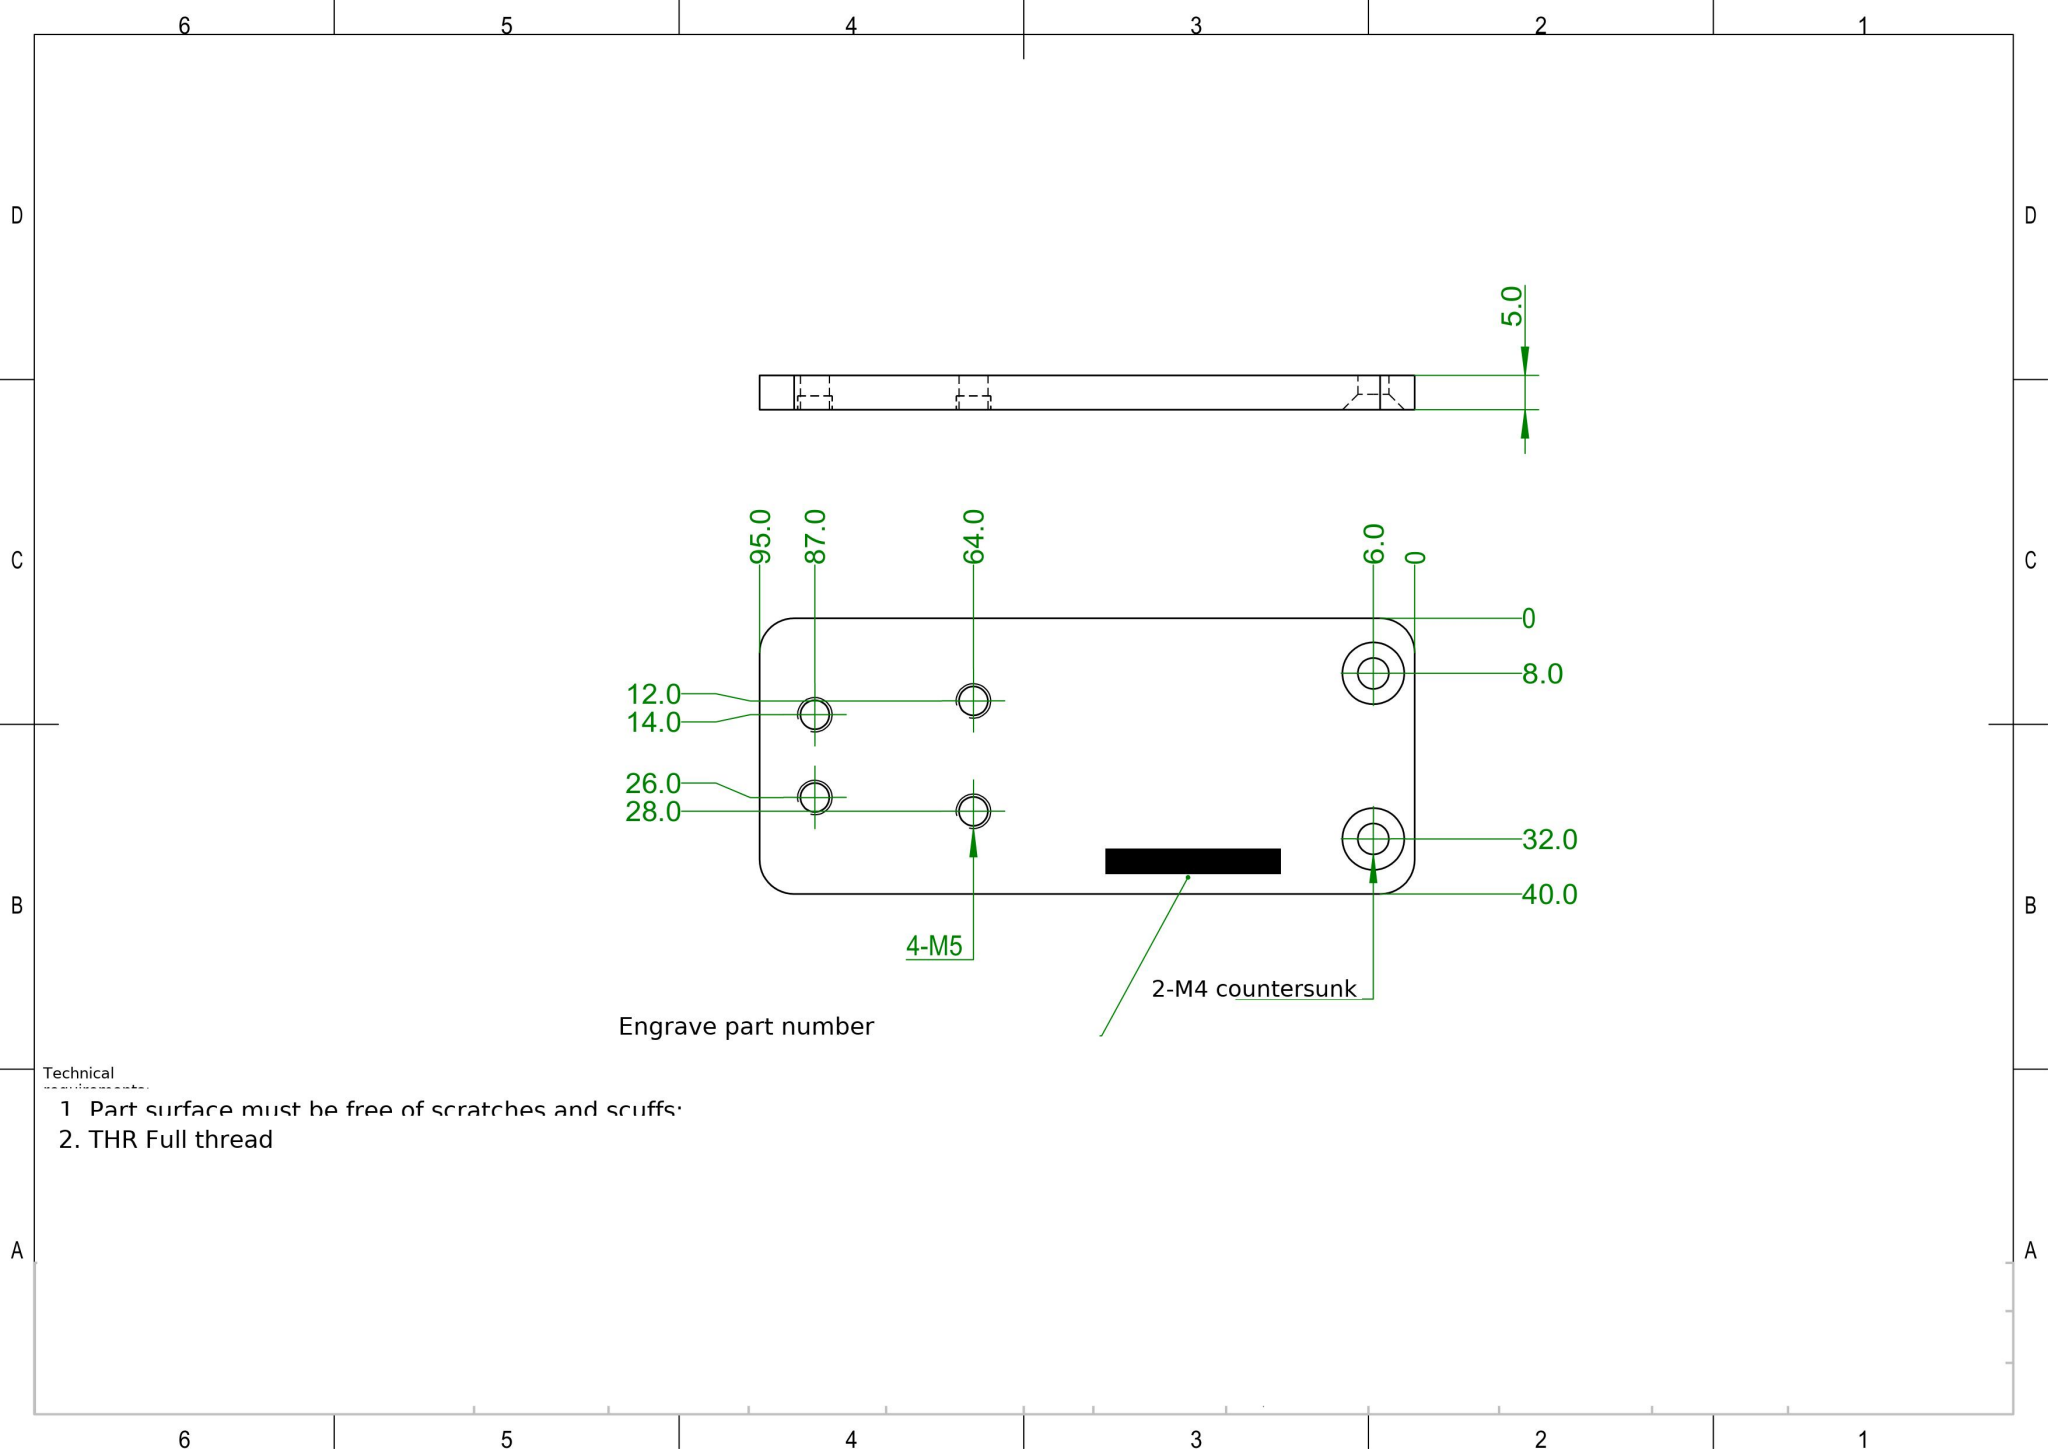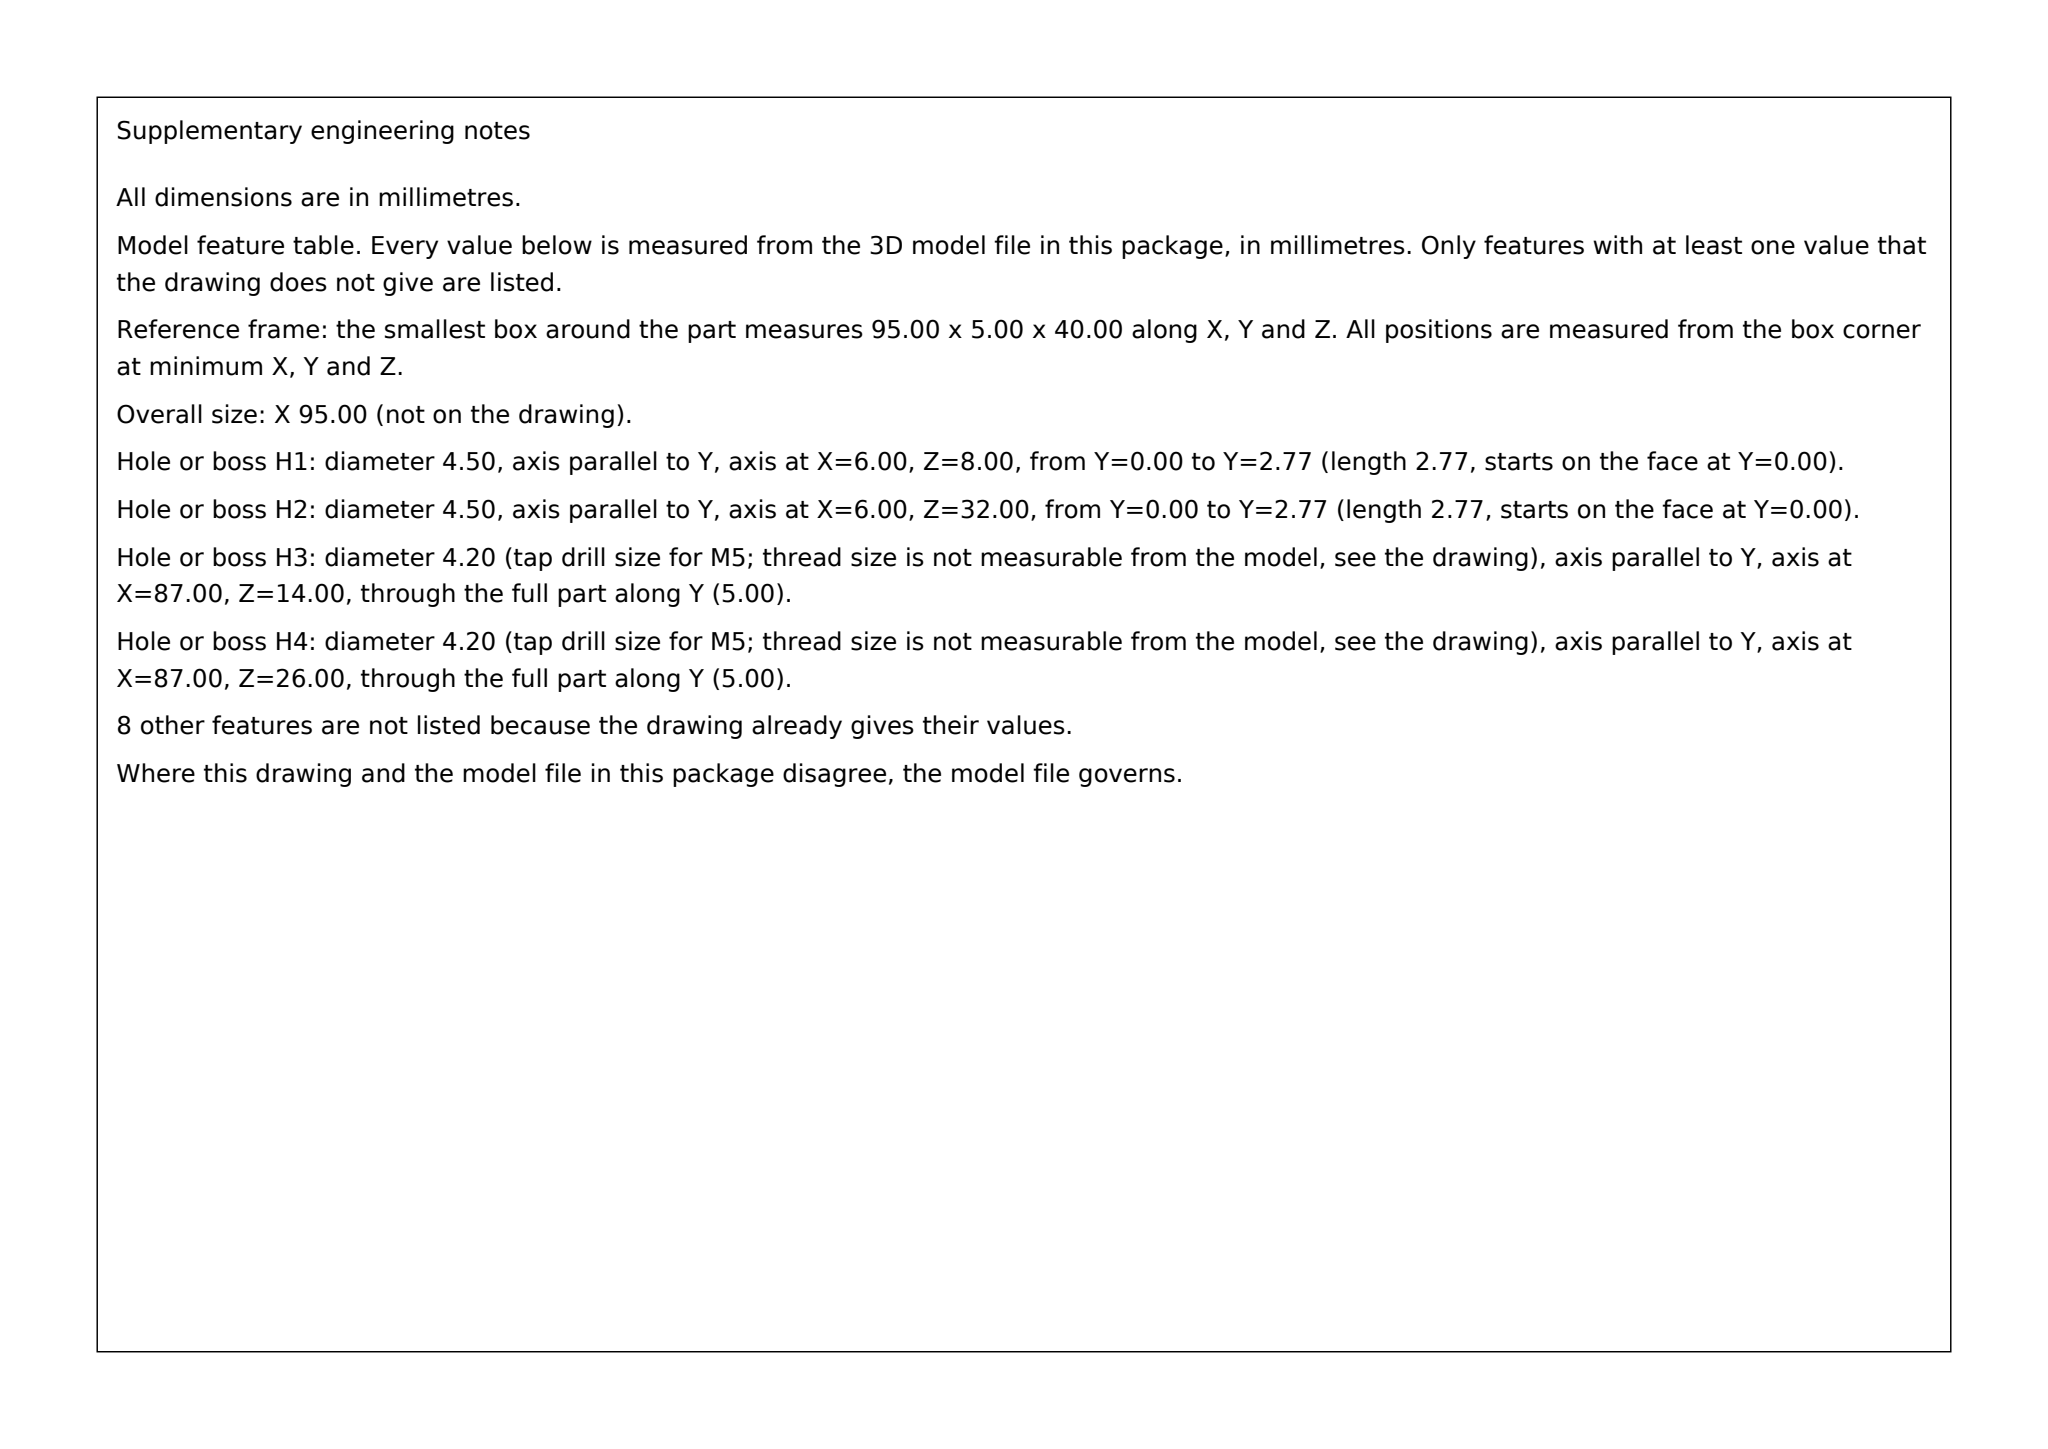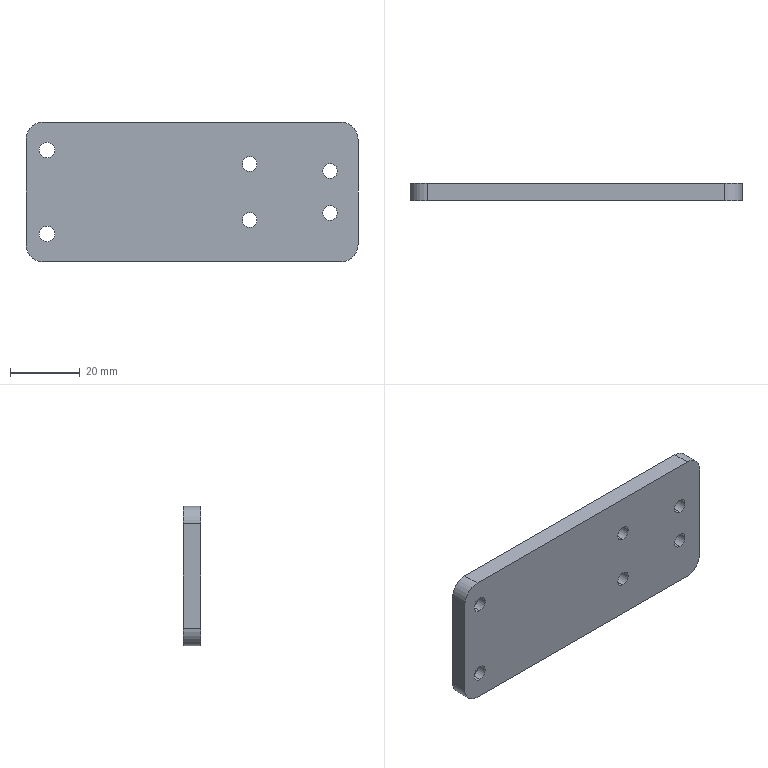Part | SolidWorks | mm | 1 solid | 26 faces | box 95 x 5 x 40 mm | volume 18363 mm3 | cylinder 16 | plane 6 | cone 4 | commonest cylinder face diameters 4.2 x8 4.5 x4 10 x4
STEP:
#1=CARTESIAN_POINT('',(6.,-2.23,-14.25));
#2=VERTEX_POINT('',#1);
#3=CARTESIAN_POINT('',(6.,-2.23,-9.75));
#4=VERTEX_POINT('',#3);
#5=CARTESIAN_POINT('',(6.,-2.23,-12.));
#6=DIRECTION('',(0.,1.,0.));
#7=DIRECTION('',(0.,0.,1.));
#8=AXIS2_PLACEMENT_3D('',#5,#6,#7);
#9=CIRCLE('',#8,2.25);
#10=EDGE_CURVE('',#2,#4,#9,.T.);
#11=ORIENTED_EDGE('',*,*,#10,.F.);
#12=CARTESIAN_POINT('',(6.,0.,-16.48));
#13=VERTEX_POINT('',#12);
#14=CARTESIAN_POINT('',(6.,0.,-16.48));
#15=DIRECTION('',(0.,0.7071,-0.7071));
#16=VECTOR('',#15,1000.);
#17=LINE('',#14,#16);
#18=EDGE_CURVE('',#2,#13,#17,.T.);
#19=ORIENTED_EDGE('',*,*,#18,.T.);
#20=CARTESIAN_POINT('',(6.,0.,-7.52));
#21=VERTEX_POINT('',#20);
#22=CARTESIAN_POINT('',(6.,0.,-12.));
#23=DIRECTION('',(0.,1.,0.));
#24=DIRECTION('',(0.,0.,1.));
#25=AXIS2_PLACEMENT_3D('',#22,#23,#24);
#26=CIRCLE('',#25,4.48);
#27=EDGE_CURVE('',#13,#21,#26,.T.);
#28=ORIENTED_EDGE('',*,*,#27,.T.);
#29=CARTESIAN_POINT('',(6.,0.,-7.52));
#30=DIRECTION('',(0.,0.7071,0.7071));
#31=VECTOR('',#30,1000.);
#32=LINE('',#29,#31);
#33=EDGE_CURVE('',#4,#21,#32,.T.);
#34=ORIENTED_EDGE('',*,*,#33,.F.);
#35=EDGE_LOOP('',(#11,#19,#28,#34));
#36=FACE_OUTER_BOUND('',#35,.T.);
#37=CARTESIAN_POINT('',(6.,0.,-12.));
#38=DIRECTION('',(0.,1.,0.));
#39=DIRECTION('',(0.,0.,1.));
#40=AXIS2_PLACEMENT_3D('',#37,#38,#39);
#41=CONICAL_SURFACE('',#40,4.48,0.7854);
#42=ADVANCED_FACE('',(#36),#41,.F.);
#43=CARTESIAN_POINT('',(6.,-5.,-14.25));
#44=VERTEX_POINT('',#43);
#45=CARTESIAN_POINT('',(6.,-5.,-9.75));
#46=VERTEX_POINT('',#45);
#47=CARTESIAN_POINT('',(6.,-5.,-12.));
#48=DIRECTION('',(0.,1.,0.));
#49=DIRECTION('',(0.,0.,1.));
#50=AXIS2_PLACEMENT_3D('',#47,#48,#49);
#51=CIRCLE('',#50,2.25);
#52=EDGE_CURVE('',#44,#46,#51,.T.);
#53=ORIENTED_EDGE('',*,*,#52,.F.);
#54=CARTESIAN_POINT('',(6.,0.,-14.25));
#55=DIRECTION('',(0.,1.,0.));
#56=VECTOR('',#55,1000.);
#57=LINE('',#54,#56);
#58=EDGE_CURVE('',#44,#2,#57,.T.);
#59=ORIENTED_EDGE('',*,*,#58,.T.);
#60=ORIENTED_EDGE('',*,*,#10,.T.);
#61=CARTESIAN_POINT('',(6.,0.,-9.75));
#62=DIRECTION('',(0.,1.,0.));
#63=VECTOR('',#62,1000.);
#64=LINE('',#61,#63);
#65=EDGE_CURVE('',#46,#4,#64,.T.);
#66=ORIENTED_EDGE('',*,*,#65,.F.);
#67=EDGE_LOOP('',(#53,#59,#60,#66));
#68=FACE_OUTER_BOUND('',#67,.T.);
#69=CARTESIAN_POINT('',(6.,0.,-12.));
#70=DIRECTION('',(0.,1.,0.));
#71=DIRECTION('',(0.,0.,1.));
#72=AXIS2_PLACEMENT_3D('',#69,#70,#71);
#73=CYLINDRICAL_SURFACE('',#72,2.25);
#74=ADVANCED_FACE('',(#68),#73,.F.);
#75=CARTESIAN_POINT('',(6.,-2.23,9.75));
#76=VERTEX_POINT('',#75);
#77=CARTESIAN_POINT('',(6.,-2.23,14.25));
#78=VERTEX_POINT('',#77);
#79=CARTESIAN_POINT('',(6.,-2.23,12.));
#80=DIRECTION('',(0.,1.,0.));
#81=DIRECTION('',(0.,0.,1.));
#82=AXIS2_PLACEMENT_3D('',#79,#80,#81);
#83=CIRCLE('',#82,2.25);
#84=EDGE_CURVE('',#76,#78,#83,.T.);
#85=ORIENTED_EDGE('',*,*,#84,.F.);
#86=CARTESIAN_POINT('',(6.,0.,7.52));
#87=VERTEX_POINT('',#86);
#88=CARTESIAN_POINT('',(6.,0.,7.52));
#89=DIRECTION('',(0.,0.7071,-0.7071));
#90=VECTOR('',#89,1000.);
#91=LINE('',#88,#90);
#92=EDGE_CURVE('',#76,#87,#91,.T.);
#93=ORIENTED_EDGE('',*,*,#92,.T.);
#94=CARTESIAN_POINT('',(6.,0.,16.48));
#95=VERTEX_POINT('',#94);
#96=CARTESIAN_POINT('',(6.,0.,12.));
#97=DIRECTION('',(0.,1.,0.));
#98=DIRECTION('',(0.,0.,1.));
#99=AXIS2_PLACEMENT_3D('',#96,#97,#98);
#100=CIRCLE('',#99,4.48);
#101=EDGE_CURVE('',#87,#95,#100,.T.);
#102=ORIENTED_EDGE('',*,*,#101,.T.);
#103=CARTESIAN_POINT('',(6.,0.,16.48));
#104=DIRECTION('',(0.,0.7071,0.7071));
#105=VECTOR('',#104,1000.);
#106=LINE('',#103,#105);
#107=EDGE_CURVE('',#78,#95,#106,.T.);
#108=ORIENTED_EDGE('',*,*,#107,.F.);
#109=EDGE_LOOP('',(#85,#93,#102,#108));
#110=FACE_OUTER_BOUND('',#109,.T.);
#111=CARTESIAN_POINT('',(6.,0.,12.));
#112=DIRECTION('',(0.,1.,0.));
#113=DIRECTION('',(0.,0.,1.));
#114=AXIS2_PLACEMENT_3D('',#111,#112,#113);
#115=CONICAL_SURFACE('',#114,4.48,0.7854);
#116=ADVANCED_FACE('',(#110),#115,.F.);
#117=CARTESIAN_POINT('',(6.,-5.,9.75));
#118=VERTEX_POINT('',#117);
#119=CARTESIAN_POINT('',(6.,-5.,14.25));
#120=VERTEX_POINT('',#119);
#121=CARTESIAN_POINT('',(6.,-5.,12.));
#122=DIRECTION('',(0.,1.,0.));
#123=DIRECTION('',(0.,0.,1.));
#124=AXIS2_PLACEMENT_3D('',#121,#122,#123);
#125=CIRCLE('',#124,2.25);
#126=EDGE_CURVE('',#118,#120,#125,.T.);
#127=ORIENTED_EDGE('',*,*,#126,.F.);
#128=CARTESIAN_POINT('',(6.,0.,9.75));
#129=DIRECTION('',(0.,1.,0.));
#130=VECTOR('',#129,1000.);
#131=LINE('',#128,#130);
#132=EDGE_CURVE('',#118,#76,#131,.T.);
#133=ORIENTED_EDGE('',*,*,#132,.T.);
#134=ORIENTED_EDGE('',*,*,#84,.T.);
#135=CARTESIAN_POINT('',(6.,0.,14.25));
#136=DIRECTION('',(0.,1.,0.));
#137=VECTOR('',#136,1000.);
#138=LINE('',#135,#137);
#139=EDGE_CURVE('',#120,#78,#138,.T.);
#140=ORIENTED_EDGE('',*,*,#139,.F.);
#141=EDGE_LOOP('',(#127,#133,#134,#140));
#142=FACE_OUTER_BOUND('',#141,.T.);
#143=CARTESIAN_POINT('',(6.,0.,12.));
#144=DIRECTION('',(0.,1.,0.));
#145=DIRECTION('',(0.,0.,1.));
#146=AXIS2_PLACEMENT_3D('',#143,#144,#145);
#147=CYLINDRICAL_SURFACE('',#146,2.25);
#148=ADVANCED_FACE('',(#142),#147,.F.);
#149=CARTESIAN_POINT('',(87.,-5.,-8.1));
#150=VERTEX_POINT('',#149);
#151=CARTESIAN_POINT('',(87.,-5.,-3.9));
#152=VERTEX_POINT('',#151);
#153=CARTESIAN_POINT('',(87.,-5.,-6.));
#154=DIRECTION('',(0.,1.,0.));
#155=DIRECTION('',(0.,0.,1.));
#156=AXIS2_PLACEMENT_3D('',#153,#154,#155);
#157=CIRCLE('',#156,2.1);
#158=EDGE_CURVE('',#150,#152,#157,.T.);
#159=ORIENTED_EDGE('',*,*,#158,.F.);
#160=CARTESIAN_POINT('',(87.,0.,-8.1));
#161=VERTEX_POINT('',#160);
#162=CARTESIAN_POINT('',(87.,0.,-8.1));
#163=DIRECTION('',(0.,1.,0.));
#164=VECTOR('',#163,1000.);
#165=LINE('',#162,#164);
#166=EDGE_CURVE('',#150,#161,#165,.T.);
#167=ORIENTED_EDGE('',*,*,#166,.T.);
#168=CARTESIAN_POINT('',(87.,0.,-3.9));
#169=VERTEX_POINT('',#168);
#170=CARTESIAN_POINT('',(87.,0.,-6.));
#171=DIRECTION('',(0.,1.,0.));
#172=DIRECTION('',(0.,0.,1.));
#173=AXIS2_PLACEMENT_3D('',#170,#171,#172);
#174=CIRCLE('',#173,2.1);
#175=EDGE_CURVE('',#161,#169,#174,.T.);
#176=ORIENTED_EDGE('',*,*,#175,.T.);
#177=CARTESIAN_POINT('',(87.,0.,-3.9));
#178=DIRECTION('',(0.,1.,0.));
#179=VECTOR('',#178,1000.);
#180=LINE('',#177,#179);
#181=EDGE_CURVE('',#152,#169,#180,.T.);
#182=ORIENTED_EDGE('',*,*,#181,.F.);
#183=EDGE_LOOP('',(#159,#167,#176,#182));
#184=FACE_OUTER_BOUND('',#183,.T.);
#185=CARTESIAN_POINT('',(87.,0.,-6.));
#186=DIRECTION('',(0.,1.,0.));
#187=DIRECTION('',(0.,0.,1.));
#188=AXIS2_PLACEMENT_3D('',#185,#186,#187);
#189=CYLINDRICAL_SURFACE('',#188,2.1);
#190=ADVANCED_FACE('',(#184),#189,.F.);
#191=CARTESIAN_POINT('',(64.,-5.,5.9));
#192=VERTEX_POINT('',#191);
#193=CARTESIAN_POINT('',(64.,-5.,10.1));
#194=VERTEX_POINT('',#193);
#195=CARTESIAN_POINT('',(64.,-5.,8.));
#196=DIRECTION('',(0.,1.,0.));
#197=DIRECTION('',(0.,0.,1.));
#198=AXIS2_PLACEMENT_3D('',#195,#196,#197);
#199=CIRCLE('',#198,2.1);
#200=EDGE_CURVE('',#192,#194,#199,.T.);
#201=ORIENTED_EDGE('',*,*,#200,.F.);
#202=CARTESIAN_POINT('',(64.,0.,5.9));
#203=VERTEX_POINT('',#202);
#204=CARTESIAN_POINT('',(64.,0.,5.9));
#205=DIRECTION('',(0.,1.,0.));
#206=VECTOR('',#205,1000.);
#207=LINE('',#204,#206);
#208=EDGE_CURVE('',#192,#203,#207,.T.);
#209=ORIENTED_EDGE('',*,*,#208,.T.);
#210=CARTESIAN_POINT('',(64.,0.,10.1));
#211=VERTEX_POINT('',#210);
#212=CARTESIAN_POINT('',(64.,0.,8.));
#213=DIRECTION('',(0.,1.,0.));
#214=DIRECTION('',(0.,0.,1.));
#215=AXIS2_PLACEMENT_3D('',#212,#213,#214);
#216=CIRCLE('',#215,2.1);
#217=EDGE_CURVE('',#203,#211,#216,.T.);
#218=ORIENTED_EDGE('',*,*,#217,.T.);
#219=CARTESIAN_POINT('',(64.,0.,10.1));
#220=DIRECTION('',(0.,1.,0.));
#221=VECTOR('',#220,1000.);
#222=LINE('',#219,#221);
#223=EDGE_CURVE('',#194,#211,#222,.T.);
#224=ORIENTED_EDGE('',*,*,#223,.F.);
#225=EDGE_LOOP('',(#201,#209,#218,#224));
#226=FACE_OUTER_BOUND('',#225,.T.);
#227=CARTESIAN_POINT('',(64.,0.,8.));
#228=DIRECTION('',(0.,1.,0.));
#229=DIRECTION('',(0.,0.,1.));
#230=AXIS2_PLACEMENT_3D('',#227,#228,#229);
#231=CYLINDRICAL_SURFACE('',#230,2.1);
#232=ADVANCED_FACE('',(#226),#231,.F.);
#233=CARTESIAN_POINT('',(87.,-5.,3.9));
#234=VERTEX_POINT('',#233);
#235=CARTESIAN_POINT('',(87.,-5.,8.1));
#236=VERTEX_POINT('',#235);
#237=CARTESIAN_POINT('',(87.,-5.,6.));
#238=DIRECTION('',(0.,1.,0.));
#239=DIRECTION('',(0.,0.,1.));
#240=AXIS2_PLACEMENT_3D('',#237,#238,#239);
#241=CIRCLE('',#240,2.1);
#242=EDGE_CURVE('',#234,#236,#241,.T.);
#243=ORIENTED_EDGE('',*,*,#242,.F.);
#244=CARTESIAN_POINT('',(87.,0.,3.9));
#245=VERTEX_POINT('',#244);
#246=CARTESIAN_POINT('',(87.,0.,3.9));
#247=DIRECTION('',(0.,1.,0.));
#248=VECTOR('',#247,1000.);
#249=LINE('',#246,#248);
#250=EDGE_CURVE('',#234,#245,#249,.T.);
#251=ORIENTED_EDGE('',*,*,#250,.T.);
#252=CARTESIAN_POINT('',(87.,0.,8.1));
#253=VERTEX_POINT('',#252);
#254=CARTESIAN_POINT('',(87.,0.,6.));
#255=DIRECTION('',(0.,1.,0.));
#256=DIRECTION('',(0.,0.,1.));
#257=AXIS2_PLACEMENT_3D('',#254,#255,#256);
#258=CIRCLE('',#257,2.1);
#259=EDGE_CURVE('',#245,#253,#258,.T.);
#260=ORIENTED_EDGE('',*,*,#259,.T.);
#261=CARTESIAN_POINT('',(87.,0.,8.1));
#262=DIRECTION('',(0.,1.,0.));
#263=VECTOR('',#262,1000.);
#264=LINE('',#261,#263);
#265=EDGE_CURVE('',#236,#253,#264,.T.);
#266=ORIENTED_EDGE('',*,*,#265,.F.);
#267=EDGE_LOOP('',(#243,#251,#260,#266));
#268=FACE_OUTER_BOUND('',#267,.T.);
#269=CARTESIAN_POINT('',(87.,0.,6.));
#270=DIRECTION('',(0.,1.,0.));
#271=DIRECTION('',(0.,0.,1.));
#272=AXIS2_PLACEMENT_3D('',#269,#270,#271);
#273=CYLINDRICAL_SURFACE('',#272,2.1);
#274=ADVANCED_FACE('',(#268),#273,.F.);
#275=CARTESIAN_POINT('',(64.,-5.,-10.1));
#276=VERTEX_POINT('',#275);
#277=CARTESIAN_POINT('',(64.,-5.,-5.9));
#278=VERTEX_POINT('',#277);
#279=CARTESIAN_POINT('',(64.,-5.,-8.));
#280=DIRECTION('',(0.,1.,0.));
#281=DIRECTION('',(0.,0.,1.));
#282=AXIS2_PLACEMENT_3D('',#279,#280,#281);
#283=CIRCLE('',#282,2.1);
#284=EDGE_CURVE('',#276,#278,#283,.T.);
#285=ORIENTED_EDGE('',*,*,#284,.F.);
#286=CARTESIAN_POINT('',(64.,0.,-10.1));
#287=VERTEX_POINT('',#286);
#288=CARTESIAN_POINT('',(64.,0.,-10.1));
#289=DIRECTION('',(0.,1.,0.));
#290=VECTOR('',#289,1000.);
#291=LINE('',#288,#290);
#292=EDGE_CURVE('',#276,#287,#291,.T.);
#293=ORIENTED_EDGE('',*,*,#292,.T.);
#294=CARTESIAN_POINT('',(64.,0.,-5.9));
#295=VERTEX_POINT('',#294);
#296=CARTESIAN_POINT('',(64.,0.,-8.));
#297=DIRECTION('',(0.,1.,0.));
#298=DIRECTION('',(0.,0.,1.));
#299=AXIS2_PLACEMENT_3D('',#296,#297,#298);
#300=CIRCLE('',#299,2.1);
#301=EDGE_CURVE('',#287,#295,#300,.T.);
#302=ORIENTED_EDGE('',*,*,#301,.T.);
#303=CARTESIAN_POINT('',(64.,0.,-5.9));
#304=DIRECTION('',(0.,1.,0.));
#305=VECTOR('',#304,1000.);
#306=LINE('',#303,#305);
#307=EDGE_CURVE('',#278,#295,#306,.T.);
#308=ORIENTED_EDGE('',*,*,#307,.F.);
#309=EDGE_LOOP('',(#285,#293,#302,#308));
#310=FACE_OUTER_BOUND('',#309,.T.);
#311=CARTESIAN_POINT('',(64.,0.,-8.));
#312=DIRECTION('',(0.,1.,0.));
#313=DIRECTION('',(0.,0.,1.));
#314=AXIS2_PLACEMENT_3D('',#311,#312,#313);
#315=CYLINDRICAL_SURFACE('',#314,2.1);
#316=ADVANCED_FACE('',(#310),#315,.F.);
#317=CARTESIAN_POINT('',(6.,-5.,-12.));
#318=DIRECTION('',(0.,1.,0.));
#319=DIRECTION('',(0.,0.,1.));
#320=AXIS2_PLACEMENT_3D('',#317,#318,#319);
#321=CIRCLE('',#320,2.25);
#322=EDGE_CURVE('',#46,#44,#321,.T.);
#323=ORIENTED_EDGE('',*,*,#322,.T.);
#324=ORIENTED_EDGE('',*,*,#52,.T.);
#325=EDGE_LOOP('',(#323,#324));
#326=FACE_BOUND('',#325,.T.);
#327=CARTESIAN_POINT('',(6.,-5.,12.));
#328=DIRECTION('',(0.,1.,0.));
#329=DIRECTION('',(0.,0.,1.));
#330=AXIS2_PLACEMENT_3D('',#327,#328,#329);
#331=CIRCLE('',#330,2.25);
#332=EDGE_CURVE('',#120,#118,#331,.T.);
#333=ORIENTED_EDGE('',*,*,#332,.T.);
#334=ORIENTED_EDGE('',*,*,#126,.T.);
#335=EDGE_LOOP('',(#333,#334));
#336=FACE_BOUND('',#335,.T.);
#337=CARTESIAN_POINT('',(87.,-5.,-6.));
#338=DIRECTION('',(0.,1.,0.));
#339=DIRECTION('',(0.,0.,1.));
#340=AXIS2_PLACEMENT_3D('',#337,#338,#339);
#341=CIRCLE('',#340,2.1);
#342=EDGE_CURVE('',#152,#150,#341,.T.);
#343=ORIENTED_EDGE('',*,*,#342,.T.);
#344=ORIENTED_EDGE('',*,*,#158,.T.);
#345=EDGE_LOOP('',(#343,#344));
#346=FACE_BOUND('',#345,.T.);
#347=CARTESIAN_POINT('',(64.,-5.,8.));
#348=DIRECTION('',(0.,1.,0.));
#349=DIRECTION('',(0.,0.,1.));
#350=AXIS2_PLACEMENT_3D('',#347,#348,#349);
#351=CIRCLE('',#350,2.1);
#352=EDGE_CURVE('',#194,#192,#351,.T.);
#353=ORIENTED_EDGE('',*,*,#352,.T.);
#354=ORIENTED_EDGE('',*,*,#200,.T.);
#355=EDGE_LOOP('',(#353,#354));
#356=FACE_BOUND('',#355,.T.);
#357=CARTESIAN_POINT('',(87.,-5.,6.));
#358=DIRECTION('',(0.,1.,0.));
#359=DIRECTION('',(0.,0.,1.));
#360=AXIS2_PLACEMENT_3D('',#357,#358,#359);
#361=CIRCLE('',#360,2.1);
#362=EDGE_CURVE('',#236,#234,#361,.T.);
#363=ORIENTED_EDGE('',*,*,#362,.T.);
#364=ORIENTED_EDGE('',*,*,#242,.T.);
#365=EDGE_LOOP('',(#363,#364));
#366=FACE_BOUND('',#365,.T.);
#367=CARTESIAN_POINT('',(64.,-5.,-8.));
#368=DIRECTION('',(0.,1.,0.));
#369=DIRECTION('',(0.,0.,1.));
#370=AXIS2_PLACEMENT_3D('',#367,#368,#369);
#371=CIRCLE('',#370,2.1);
#372=EDGE_CURVE('',#278,#276,#371,.T.);
#373=ORIENTED_EDGE('',*,*,#372,.T.);
#374=ORIENTED_EDGE('',*,*,#284,.T.);
#375=EDGE_LOOP('',(#373,#374));
#376=FACE_BOUND('',#375,.T.);
#377=CARTESIAN_POINT('',(5.,-5.,-20.));
#378=VERTEX_POINT('',#377);
#379=CARTESIAN_POINT('',(90.,-5.,-20.));
#380=VERTEX_POINT('',#379);
#381=CARTESIAN_POINT('',(0.,-5.,-20.));
#382=DIRECTION('',(1.,0.,0.));
#383=VECTOR('',#382,1000.);
#384=LINE('',#381,#383);
#385=EDGE_CURVE('',#378,#380,#384,.T.);
#386=ORIENTED_EDGE('',*,*,#385,.T.);
#387=CARTESIAN_POINT('',(95.,-5.,-15.));
#388=VERTEX_POINT('',#387);
#389=CARTESIAN_POINT('',(90.,-5.,-15.));
#390=DIRECTION('',(0.,-1.,0.));
#391=DIRECTION('',(0.,0.,1.));
#392=AXIS2_PLACEMENT_3D('',#389,#390,#391);
#393=CIRCLE('',#392,5.);
#394=EDGE_CURVE('',#380,#388,#393,.T.);
#395=ORIENTED_EDGE('',*,*,#394,.T.);
#396=CARTESIAN_POINT('',(95.,-5.,15.));
#397=VERTEX_POINT('',#396);
#398=CARTESIAN_POINT('',(95.,-5.,20.));
#399=DIRECTION('',(0.,0.,-1.));
#400=VECTOR('',#399,1000.);
#401=LINE('',#398,#400);
#402=EDGE_CURVE('',#397,#388,#401,.T.);
#403=ORIENTED_EDGE('',*,*,#402,.F.);
#404=CARTESIAN_POINT('',(90.,-5.,20.));
#405=VERTEX_POINT('',#404);
#406=CARTESIAN_POINT('',(90.,-5.,15.));
#407=DIRECTION('',(0.,-1.,0.));
#408=DIRECTION('',(0.,0.,1.));
#409=AXIS2_PLACEMENT_3D('',#406,#407,#408);
#410=CIRCLE('',#409,5.);
#411=EDGE_CURVE('',#397,#405,#410,.T.);
#412=ORIENTED_EDGE('',*,*,#411,.T.);
#413=CARTESIAN_POINT('',(5.,-5.,20.));
#414=VERTEX_POINT('',#413);
#415=CARTESIAN_POINT('',(0.,-5.,20.));
#416=DIRECTION('',(1.,0.,0.));
#417=VECTOR('',#416,1000.);
#418=LINE('',#415,#417);
#419=EDGE_CURVE('',#414,#405,#418,.T.);
#420=ORIENTED_EDGE('',*,*,#419,.F.);
#421=CARTESIAN_POINT('',(0.,-5.,15.));
#422=VERTEX_POINT('',#421);
#423=CARTESIAN_POINT('',(5.,-5.,15.));
#424=DIRECTION('',(0.,-1.,0.));
#425=DIRECTION('',(0.,0.,1.));
#426=AXIS2_PLACEMENT_3D('',#423,#424,#425);
#427=CIRCLE('',#426,5.);
#428=EDGE_CURVE('',#414,#422,#427,.T.);
#429=ORIENTED_EDGE('',*,*,#428,.T.);
#430=CARTESIAN_POINT('',(0.,-5.,-15.));
#431=VERTEX_POINT('',#430);
#432=CARTESIAN_POINT('',(0.,-5.,20.));
#433=DIRECTION('',(0.,0.,-1.));
#434=VECTOR('',#433,1000.);
#435=LINE('',#432,#434);
#436=EDGE_CURVE('',#422,#431,#435,.T.);
#437=ORIENTED_EDGE('',*,*,#436,.T.);
#438=CARTESIAN_POINT('',(5.,-5.,-15.));
#439=DIRECTION('',(0.,-1.,0.));
#440=DIRECTION('',(0.,0.,1.));
#441=AXIS2_PLACEMENT_3D('',#438,#439,#440);
#442=CIRCLE('',#441,5.);
#443=EDGE_CURVE('',#431,#378,#442,.T.);
#444=ORIENTED_EDGE('',*,*,#443,.T.);
#445=EDGE_LOOP('',(#386,#395,#403,#412,#420,#429,#437,#444));
#446=FACE_OUTER_BOUND('',#445,.T.);
#447=CARTESIAN_POINT('',(0.,-5.,20.));
#448=DIRECTION('',(0.,1.,0.));
#449=DIRECTION('',(0.,0.,1.));
#450=AXIS2_PLACEMENT_3D('',#447,#448,#449);
#451=PLANE('',#450);
#452=ADVANCED_FACE('',(#326,#336,#346,#356,#366,#376,#446),#451,.F.);
#453=ORIENTED_EDGE('',*,*,#402,.T.);
#454=CARTESIAN_POINT('',(95.,0.,-15.));
#455=VERTEX_POINT('',#454);
#456=CARTESIAN_POINT('',(95.,0.,-15.));
#457=DIRECTION('',(0.,1.,0.));
#458=VECTOR('',#457,1000.);
#459=LINE('',#456,#458);
#460=EDGE_CURVE('',#388,#455,#459,.T.);
#461=ORIENTED_EDGE('',*,*,#460,.T.);
#462=CARTESIAN_POINT('',(95.,0.,15.));
#463=VERTEX_POINT('',#462);
#464=CARTESIAN_POINT('',(95.,0.,20.));
#465=DIRECTION('',(0.,0.,-1.));
#466=VECTOR('',#465,1000.);
#467=LINE('',#464,#466);
#468=EDGE_CURVE('',#463,#455,#467,.T.);
#469=ORIENTED_EDGE('',*,*,#468,.F.);
#470=CARTESIAN_POINT('',(95.,-5.,15.));
#471=DIRECTION('',(0.,-1.,0.));
#472=VECTOR('',#471,1000.);
#473=LINE('',#470,#472);
#474=EDGE_CURVE('',#463,#397,#473,.T.);
#475=ORIENTED_EDGE('',*,*,#474,.T.);
#476=EDGE_LOOP('',(#453,#461,#469,#475));
#477=FACE_OUTER_BOUND('',#476,.T.);
#478=CARTESIAN_POINT('',(95.,0.,20.));
#479=DIRECTION('',(1.,0.,0.));
#480=DIRECTION('',(0.,0.,-1.));
#481=AXIS2_PLACEMENT_3D('',#478,#479,#480);
#482=PLANE('',#481);
#483=ADVANCED_FACE('',(#477),#482,.T.);
#484=CARTESIAN_POINT('',(6.,0.,-12.));
#485=DIRECTION('',(0.,1.,0.));
#486=DIRECTION('',(0.,0.,1.));
#487=AXIS2_PLACEMENT_3D('',#484,#485,#486);
#488=CIRCLE('',#487,4.48);
#489=EDGE_CURVE('',#21,#13,#488,.T.);
#490=ORIENTED_EDGE('',*,*,#489,.F.);
#491=ORIENTED_EDGE('',*,*,#27,.F.);
#492=EDGE_LOOP('',(#490,#491));
#493=FACE_BOUND('',#492,.T.);
#494=CARTESIAN_POINT('',(6.,0.,12.));
#495=DIRECTION('',(0.,1.,0.));
#496=DIRECTION('',(0.,0.,1.));
#497=AXIS2_PLACEMENT_3D('',#494,#495,#496);
#498=CIRCLE('',#497,4.48);
#499=EDGE_CURVE('',#95,#87,#498,.T.);
#500=ORIENTED_EDGE('',*,*,#499,.F.);
#501=ORIENTED_EDGE('',*,*,#101,.F.);
#502=EDGE_LOOP('',(#500,#501));
#503=FACE_BOUND('',#502,.T.);
#504=CARTESIAN_POINT('',(87.,0.,-6.));
#505=DIRECTION('',(0.,1.,0.));
#506=DIRECTION('',(0.,0.,1.));
#507=AXIS2_PLACEMENT_3D('',#504,#505,#506);
#508=CIRCLE('',#507,2.1);
#509=EDGE_CURVE('',#169,#161,#508,.T.);
#510=ORIENTED_EDGE('',*,*,#509,.F.);
#511=ORIENTED_EDGE('',*,*,#175,.F.);
#512=EDGE_LOOP('',(#510,#511));
#513=FACE_BOUND('',#512,.T.);
#514=CARTESIAN_POINT('',(64.,0.,8.));
#515=DIRECTION('',(0.,1.,0.));
#516=DIRECTION('',(0.,0.,1.));
#517=AXIS2_PLACEMENT_3D('',#514,#515,#516);
#518=CIRCLE('',#517,2.1);
#519=EDGE_CURVE('',#211,#203,#518,.T.);
#520=ORIENTED_EDGE('',*,*,#519,.F.);
#521=ORIENTED_EDGE('',*,*,#217,.F.);
#522=EDGE_LOOP('',(#520,#521));
#523=FACE_BOUND('',#522,.T.);
#524=CARTESIAN_POINT('',(87.,0.,6.));
#525=DIRECTION('',(0.,1.,0.));
#526=DIRECTION('',(0.,0.,1.));
#527=AXIS2_PLACEMENT_3D('',#524,#525,#526);
#528=CIRCLE('',#527,2.1);
#529=EDGE_CURVE('',#253,#245,#528,.T.);
#530=ORIENTED_EDGE('',*,*,#529,.F.);
#531=ORIENTED_EDGE('',*,*,#259,.F.);
#532=EDGE_LOOP('',(#530,#531));
#533=FACE_BOUND('',#532,.T.);
#534=CARTESIAN_POINT('',(64.,0.,-8.));
#535=DIRECTION('',(0.,1.,0.));
#536=DIRECTION('',(0.,0.,1.));
#537=AXIS2_PLACEMENT_3D('',#534,#535,#536);
#538=CIRCLE('',#537,2.1);
#539=EDGE_CURVE('',#295,#287,#538,.T.);
#540=ORIENTED_EDGE('',*,*,#539,.F.);
#541=ORIENTED_EDGE('',*,*,#301,.F.);
#542=EDGE_LOOP('',(#540,#541));
#543=FACE_BOUND('',#542,.T.);
#544=ORIENTED_EDGE('',*,*,#468,.T.);
#545=CARTESIAN_POINT('',(90.,0.,-20.));
#546=VERTEX_POINT('',#545);
#547=CARTESIAN_POINT('',(90.,0.,-15.));
#548=DIRECTION('',(0.,1.,0.));
#549=DIRECTION('',(0.,0.,1.));
#550=AXIS2_PLACEMENT_3D('',#547,#548,#549);
#551=CIRCLE('',#550,5.);
#552=EDGE_CURVE('',#455,#546,#551,.T.);
#553=ORIENTED_EDGE('',*,*,#552,.T.);
#554=CARTESIAN_POINT('',(5.,0.,-20.));
#555=VERTEX_POINT('',#554);
#556=CARTESIAN_POINT('',(0.,0.,-20.));
#557=DIRECTION('',(1.,0.,0.));
#558=VECTOR('',#557,1000.);
#559=LINE('',#556,#558);
#560=EDGE_CURVE('',#555,#546,#559,.T.);
#561=ORIENTED_EDGE('',*,*,#560,.F.);
#562=CARTESIAN_POINT('',(0.,0.,-15.));
#563=VERTEX_POINT('',#562);
#564=CARTESIAN_POINT('',(5.,0.,-15.));
#565=DIRECTION('',(0.,1.,0.));
#566=DIRECTION('',(0.,0.,1.));
#567=AXIS2_PLACEMENT_3D('',#564,#565,#566);
#568=CIRCLE('',#567,5.);
#569=EDGE_CURVE('',#555,#563,#568,.T.);
#570=ORIENTED_EDGE('',*,*,#569,.T.);
#571=CARTESIAN_POINT('',(0.,0.,15.));
#572=VERTEX_POINT('',#571);
#573=CARTESIAN_POINT('',(0.,0.,20.));
#574=DIRECTION('',(0.,0.,-1.));
#575=VECTOR('',#574,1000.);
#576=LINE('',#573,#575);
#577=EDGE_CURVE('',#572,#563,#576,.T.);
#578=ORIENTED_EDGE('',*,*,#577,.F.);
#579=CARTESIAN_POINT('',(5.,0.,20.));
#580=VERTEX_POINT('',#579);
#581=CARTESIAN_POINT('',(5.,0.,15.));
#582=DIRECTION('',(0.,1.,0.));
#583=DIRECTION('',(0.,0.,1.));
#584=AXIS2_PLACEMENT_3D('',#581,#582,#583);
#585=CIRCLE('',#584,5.);
#586=EDGE_CURVE('',#572,#580,#585,.T.);
#587=ORIENTED_EDGE('',*,*,#586,.T.);
#588=CARTESIAN_POINT('',(90.,0.,20.));
#589=VERTEX_POINT('',#588);
#590=CARTESIAN_POINT('',(0.,0.,20.));
#591=DIRECTION('',(1.,0.,0.));
#592=VECTOR('',#591,1000.);
#593=LINE('',#590,#592);
#594=EDGE_CURVE('',#580,#589,#593,.T.);
#595=ORIENTED_EDGE('',*,*,#594,.T.);
#596=CARTESIAN_POINT('',(90.,0.,15.));
#597=DIRECTION('',(0.,1.,0.));
#598=DIRECTION('',(0.,0.,1.));
#599=AXIS2_PLACEMENT_3D('',#596,#597,#598);
#600=CIRCLE('',#599,5.);
#601=EDGE_CURVE('',#589,#463,#600,.T.);
#602=ORIENTED_EDGE('',*,*,#601,.T.);
#603=EDGE_LOOP('',(#544,#553,#561,#570,#578,#587,#595,#602));
#604=FACE_OUTER_BOUND('',#603,.T.);
#605=CARTESIAN_POINT('',(0.,0.,20.));
#606=DIRECTION('',(0.,1.,0.));
#607=DIRECTION('',(0.,0.,1.));
#608=AXIS2_PLACEMENT_3D('',#605,#606,#607);
#609=PLANE('',#608);
#610=ADVANCED_FACE('',(#493,#503,#513,#523,#533,#543,#604),#609,.T.);
#611=ORIENTED_EDGE('',*,*,#577,.T.);
#612=CARTESIAN_POINT('',(0.,-5.,-15.));
#613=DIRECTION('',(0.,-1.,0.));
#614=VECTOR('',#613,1000.);
#615=LINE('',#612,#614);
#616=EDGE_CURVE('',#563,#431,#615,.T.);
#617=ORIENTED_EDGE('',*,*,#616,.T.);
#618=ORIENTED_EDGE('',*,*,#436,.F.);
#619=CARTESIAN_POINT('',(0.,0.,15.));
#620=DIRECTION('',(0.,1.,0.));
#621=VECTOR('',#620,1000.);
#622=LINE('',#619,#621);
#623=EDGE_CURVE('',#422,#572,#622,.T.);
#624=ORIENTED_EDGE('',*,*,#623,.T.);
#625=EDGE_LOOP('',(#611,#617,#618,#624));
#626=FACE_OUTER_BOUND('',#625,.T.);
#627=CARTESIAN_POINT('',(0.,-5.,20.));
#628=DIRECTION('',(-1.,0.,0.));
#629=DIRECTION('',(0.,0.,1.));
#630=AXIS2_PLACEMENT_3D('',#627,#628,#629);
#631=PLANE('',#630);
#632=ADVANCED_FACE('',(#626),#631,.T.);
#633=ORIENTED_EDGE('',*,*,#419,.T.);
#634=CARTESIAN_POINT('',(90.,0.,20.));
#635=DIRECTION('',(0.,1.,0.));
#636=VECTOR('',#635,1000.);
#637=LINE('',#634,#636);
#638=EDGE_CURVE('',#405,#589,#637,.T.);
#639=ORIENTED_EDGE('',*,*,#638,.T.);
#640=ORIENTED_EDGE('',*,*,#594,.F.);
#641=CARTESIAN_POINT('',(5.,-5.,20.));
#642=DIRECTION('',(0.,-1.,0.));
#643=VECTOR('',#642,1000.);
#644=LINE('',#641,#643);
#645=EDGE_CURVE('',#580,#414,#644,.T.);
#646=ORIENTED_EDGE('',*,*,#645,.T.);
#647=EDGE_LOOP('',(#633,#639,#640,#646));
#648=FACE_OUTER_BOUND('',#647,.T.);
#649=CARTESIAN_POINT('',(0.,0.,20.));
#650=DIRECTION('',(0.,0.,-1.));
#651=DIRECTION('',(-1.,0.,0.));
#652=AXIS2_PLACEMENT_3D('',#649,#650,#651);
#653=PLANE('',#652);
#654=ADVANCED_FACE('',(#648),#653,.F.);
#655=ORIENTED_EDGE('',*,*,#560,.T.);
#656=CARTESIAN_POINT('',(90.,0.,-20.));
#657=DIRECTION('',(0.,-1.,0.));
#658=VECTOR('',#657,1000.);
#659=LINE('',#656,#658);
#660=EDGE_CURVE('',#546,#380,#659,.T.);
#661=ORIENTED_EDGE('',*,*,#660,.T.);
#662=ORIENTED_EDGE('',*,*,#385,.F.);
#663=CARTESIAN_POINT('',(5.,0.,-20.));
#664=DIRECTION('',(0.,1.,0.));
#665=VECTOR('',#664,1000.);
#666=LINE('',#663,#665);
#667=EDGE_CURVE('',#378,#555,#666,.T.);
#668=ORIENTED_EDGE('',*,*,#667,.T.);
#669=EDGE_LOOP('',(#655,#661,#662,#668));
#670=FACE_OUTER_BOUND('',#669,.T.);
#671=CARTESIAN_POINT('',(0.,0.,-20.));
#672=DIRECTION('',(0.,0.,-1.));
#673=DIRECTION('',(-1.,0.,0.));
#674=AXIS2_PLACEMENT_3D('',#671,#672,#673);
#675=PLANE('',#674);
#676=ADVANCED_FACE('',(#670),#675,.T.);
#677=ORIENTED_EDGE('',*,*,#292,.F.);
#678=ORIENTED_EDGE('',*,*,#372,.F.);
#679=ORIENTED_EDGE('',*,*,#307,.T.);
#680=ORIENTED_EDGE('',*,*,#539,.T.);
#681=EDGE_LOOP('',(#677,#678,#679,#680));
#682=FACE_OUTER_BOUND('',#681,.T.);
#683=CARTESIAN_POINT('',(64.,0.,-8.));
#684=DIRECTION('',(0.,1.,0.));
#685=DIRECTION('',(0.,0.,1.));
#686=AXIS2_PLACEMENT_3D('',#683,#684,#685);
#687=CYLINDRICAL_SURFACE('',#686,2.1);
#688=ADVANCED_FACE('',(#682),#687,.F.);
#689=ORIENTED_EDGE('',*,*,#250,.F.);
#690=ORIENTED_EDGE('',*,*,#362,.F.);
#691=ORIENTED_EDGE('',*,*,#265,.T.);
#692=ORIENTED_EDGE('',*,*,#529,.T.);
#693=EDGE_LOOP('',(#689,#690,#691,#692));
#694=FACE_OUTER_BOUND('',#693,.T.);
#695=CARTESIAN_POINT('',(87.,0.,6.));
#696=DIRECTION('',(0.,1.,0.));
#697=DIRECTION('',(0.,0.,1.));
#698=AXIS2_PLACEMENT_3D('',#695,#696,#697);
#699=CYLINDRICAL_SURFACE('',#698,2.1);
#700=ADVANCED_FACE('',(#694),#699,.F.);
#701=ORIENTED_EDGE('',*,*,#208,.F.);
#702=ORIENTED_EDGE('',*,*,#352,.F.);
#703=ORIENTED_EDGE('',*,*,#223,.T.);
#704=ORIENTED_EDGE('',*,*,#519,.T.);
#705=EDGE_LOOP('',(#701,#702,#703,#704));
#706=FACE_OUTER_BOUND('',#705,.T.);
#707=CARTESIAN_POINT('',(64.,0.,8.));
#708=DIRECTION('',(0.,1.,0.));
#709=DIRECTION('',(0.,0.,1.));
#710=AXIS2_PLACEMENT_3D('',#707,#708,#709);
#711=CYLINDRICAL_SURFACE('',#710,2.1);
#712=ADVANCED_FACE('',(#706),#711,.F.);
#713=ORIENTED_EDGE('',*,*,#166,.F.);
#714=ORIENTED_EDGE('',*,*,#342,.F.);
#715=ORIENTED_EDGE('',*,*,#181,.T.);
#716=ORIENTED_EDGE('',*,*,#509,.T.);
#717=EDGE_LOOP('',(#713,#714,#715,#716));
#718=FACE_OUTER_BOUND('',#717,.T.);
#719=CARTESIAN_POINT('',(87.,0.,-6.));
#720=DIRECTION('',(0.,1.,0.));
#721=DIRECTION('',(0.,0.,1.));
#722=AXIS2_PLACEMENT_3D('',#719,#720,#721);
#723=CYLINDRICAL_SURFACE('',#722,2.1);
#724=ADVANCED_FACE('',(#718),#723,.F.);
#725=ORIENTED_EDGE('',*,*,#132,.F.);
#726=ORIENTED_EDGE('',*,*,#332,.F.);
#727=ORIENTED_EDGE('',*,*,#139,.T.);
#728=CARTESIAN_POINT('',(6.,-2.23,12.));
#729=DIRECTION('',(0.,1.,0.));
#730=DIRECTION('',(0.,0.,1.));
#731=AXIS2_PLACEMENT_3D('',#728,#729,#730);
#732=CIRCLE('',#731,2.25);
#733=EDGE_CURVE('',#78,#76,#732,.T.);
#734=ORIENTED_EDGE('',*,*,#733,.T.);
#735=EDGE_LOOP('',(#725,#726,#727,#734));
#736=FACE_OUTER_BOUND('',#735,.T.);
#737=CARTESIAN_POINT('',(6.,0.,12.));
#738=DIRECTION('',(0.,1.,0.));
#739=DIRECTION('',(0.,0.,1.));
#740=AXIS2_PLACEMENT_3D('',#737,#738,#739);
#741=CYLINDRICAL_SURFACE('',#740,2.25);
#742=ADVANCED_FACE('',(#736),#741,.F.);
#743=ORIENTED_EDGE('',*,*,#92,.F.);
#744=ORIENTED_EDGE('',*,*,#733,.F.);
#745=ORIENTED_EDGE('',*,*,#107,.T.);
#746=ORIENTED_EDGE('',*,*,#499,.T.);
#747=EDGE_LOOP('',(#743,#744,#745,#746));
#748=FACE_OUTER_BOUND('',#747,.T.);
#749=CARTESIAN_POINT('',(6.,0.,12.));
#750=DIRECTION('',(0.,1.,0.));
#751=DIRECTION('',(0.,0.,1.));
#752=AXIS2_PLACEMENT_3D('',#749,#750,#751);
#753=CONICAL_SURFACE('',#752,4.48,0.7854);
#754=ADVANCED_FACE('',(#748),#753,.F.);
#755=ORIENTED_EDGE('',*,*,#58,.F.);
#756=ORIENTED_EDGE('',*,*,#322,.F.);
#757=ORIENTED_EDGE('',*,*,#65,.T.);
#758=CARTESIAN_POINT('',(6.,-2.23,-12.));
#759=DIRECTION('',(0.,1.,0.));
#760=DIRECTION('',(0.,0.,1.));
#761=AXIS2_PLACEMENT_3D('',#758,#759,#760);
#762=CIRCLE('',#761,2.25);
#763=EDGE_CURVE('',#4,#2,#762,.T.);
#764=ORIENTED_EDGE('',*,*,#763,.T.);
#765=EDGE_LOOP('',(#755,#756,#757,#764));
#766=FACE_OUTER_BOUND('',#765,.T.);
#767=CARTESIAN_POINT('',(6.,0.,-12.));
#768=DIRECTION('',(0.,1.,0.));
#769=DIRECTION('',(0.,0.,1.));
#770=AXIS2_PLACEMENT_3D('',#767,#768,#769);
#771=CYLINDRICAL_SURFACE('',#770,2.25);
#772=ADVANCED_FACE('',(#766),#771,.F.);
#773=ORIENTED_EDGE('',*,*,#18,.F.);
#774=ORIENTED_EDGE('',*,*,#763,.F.);
#775=ORIENTED_EDGE('',*,*,#33,.T.);
#776=ORIENTED_EDGE('',*,*,#489,.T.);
#777=EDGE_LOOP('',(#773,#774,#775,#776));
#778=FACE_OUTER_BOUND('',#777,.T.);
#779=CARTESIAN_POINT('',(6.,0.,-12.));
#780=DIRECTION('',(0.,1.,0.));
#781=DIRECTION('',(0.,0.,1.));
#782=AXIS2_PLACEMENT_3D('',#779,#780,#781);
#783=CONICAL_SURFACE('',#782,4.48,0.7854);
#784=ADVANCED_FACE('',(#778),#783,.F.);
#785=ORIENTED_EDGE('',*,*,#552,.F.);
#786=ORIENTED_EDGE('',*,*,#460,.F.);
#787=ORIENTED_EDGE('',*,*,#394,.F.);
#788=ORIENTED_EDGE('',*,*,#660,.F.);
#789=EDGE_LOOP('',(#785,#786,#787,#788));
#790=FACE_OUTER_BOUND('',#789,.T.);
#791=CARTESIAN_POINT('',(90.,0.,-15.));
#792=DIRECTION('',(0.,-1.,0.));
#793=DIRECTION('',(0.,0.,-1.));
#794=AXIS2_PLACEMENT_3D('',#791,#792,#793);
#795=CYLINDRICAL_SURFACE('',#794,5.);
#796=ADVANCED_FACE('',(#790),#795,.T.);
#797=ORIENTED_EDGE('',*,*,#601,.F.);
#798=ORIENTED_EDGE('',*,*,#638,.F.);
#799=ORIENTED_EDGE('',*,*,#411,.F.);
#800=ORIENTED_EDGE('',*,*,#474,.F.);
#801=EDGE_LOOP('',(#797,#798,#799,#800));
#802=FACE_OUTER_BOUND('',#801,.T.);
#803=CARTESIAN_POINT('',(90.,0.,15.));
#804=DIRECTION('',(0.,1.,0.));
#805=DIRECTION('',(0.,0.,1.));
#806=AXIS2_PLACEMENT_3D('',#803,#804,#805);
#807=CYLINDRICAL_SURFACE('',#806,5.);
#808=ADVANCED_FACE('',(#802),#807,.T.);
#809=ORIENTED_EDGE('',*,*,#443,.F.);
#810=ORIENTED_EDGE('',*,*,#616,.F.);
#811=ORIENTED_EDGE('',*,*,#569,.F.);
#812=ORIENTED_EDGE('',*,*,#667,.F.);
#813=EDGE_LOOP('',(#809,#810,#811,#812));
#814=FACE_OUTER_BOUND('',#813,.T.);
#815=CARTESIAN_POINT('',(5.,0.,-15.));
#816=DIRECTION('',(0.,1.,0.));
#817=DIRECTION('',(0.,0.,1.));
#818=AXIS2_PLACEMENT_3D('',#815,#816,#817);
#819=CYLINDRICAL_SURFACE('',#818,5.);
#820=ADVANCED_FACE('',(#814),#819,.T.);
#821=ORIENTED_EDGE('',*,*,#428,.F.);
#822=ORIENTED_EDGE('',*,*,#645,.F.);
#823=ORIENTED_EDGE('',*,*,#586,.F.);
#824=ORIENTED_EDGE('',*,*,#623,.F.);
#825=EDGE_LOOP('',(#821,#822,#823,#824));
#826=FACE_OUTER_BOUND('',#825,.T.);
#827=CARTESIAN_POINT('',(5.,-5.,15.));
#828=DIRECTION('',(0.,-1.,0.));
#829=DIRECTION('',(0.,0.,-1.));
#830=AXIS2_PLACEMENT_3D('',#827,#828,#829);
#831=CYLINDRICAL_SURFACE('',#830,5.);
#832=ADVANCED_FACE('',(#826),#831,.T.);
#833=CLOSED_SHELL('',(#42,#74,#116,#148,#190,#232,#274,#316,#452,#483,#610,#632,#654,#676,#688,#700,#712,#724,#742,#754,#772,#784,#796,#808,#820,#832));
#834=MANIFOLD_SOLID_BREP('',#833);
#835=CARTESIAN_POINT('',(0.,0.,0.));
#836=DIRECTION('',(0.,0.,1.));
#837=DIRECTION('',(1.,0.,0.));
#838=AXIS2_PLACEMENT_3D('',#835,#836,#837);
#839=(LENGTH_UNIT()NAMED_UNIT(*)SI_UNIT(.MILLI.,.METRE.));
#840=UNCERTAINTY_MEASURE_WITH_UNIT(LENGTH_MEASURE(0.00001),#839,'','');
#841=(NAMED_UNIT(*)PLANE_ANGLE_UNIT()SI_UNIT($,.RADIAN.));
#842=(NAMED_UNIT(*)SI_UNIT($,.STERADIAN.)SOLID_ANGLE_UNIT());
#843=(GEOMETRIC_REPRESENTATION_CONTEXT(3)GLOBAL_UNCERTAINTY_ASSIGNED_CONTEXT((#840))GLOBAL_UNIT_ASSIGNED_CONTEXT((#839,#841,#842))REPRESENTATION_CONTEXT('',''));
#844=ADVANCED_BREP_SHAPE_REPRESENTATION('',(#834,#838),#843);